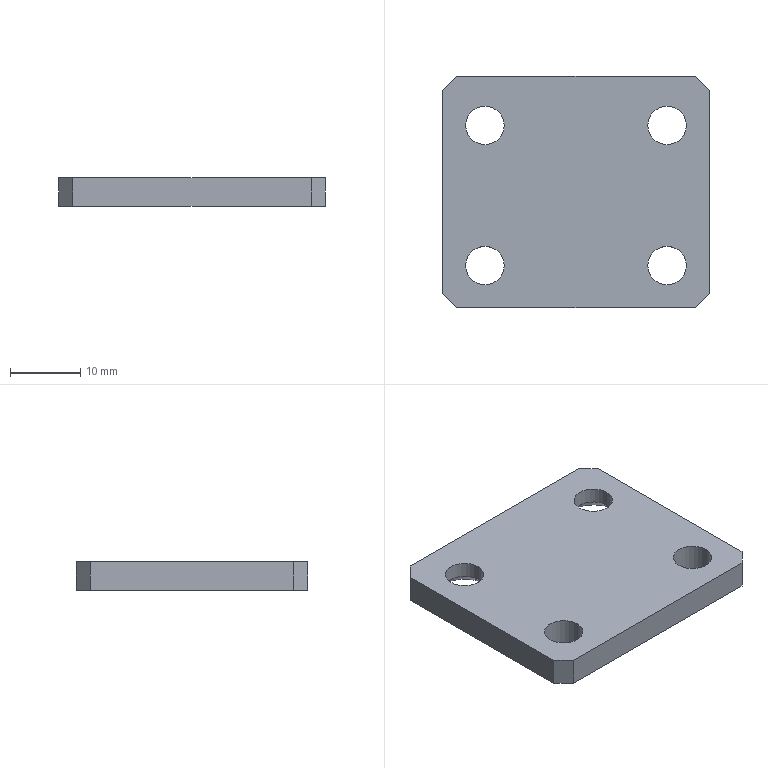Component | SolidWorks | DZ.KX.203-TC1505-30-09-01-05-20-1 | 1 solid | 22 faces | box 38 x 33 x 4 mm | volume 4540 mm3 | plane 10 | cylinder 8 | cone 4 | commonest cylinder face diameters 5.5 x8
build123d program:
from build123d import *

# Parameters (mm, degrees)
SKETCH1_W                                    = 38
SKETCH1_H                                    = 33
BOSS_EXTRUDE1_DEPTH                          = 4
HOLE_SIZE_SLOTTED_RAISED_COUNTERSUNK_2_COUNT = 2
HOLE_SIZE_SLOTTED_RAISED_COUNTERSUNK_2_PITCH = 26
F_5_5_5_5_DIAMETER_HOLE1_D                   = 5.5
CHAMFER1_SIZE                                = 2


with BuildPart() as part:
    # Sketch1 → Boss-Extrude1 (new body)
    with BuildSketch(Plane.XY):
        Rectangle(SKETCH1_W, SKETCH1_H)
    extrude(amount=BOSS_EXTRUDE1_DEPTH)

    # Sketch2 → Hole Size Slotted Raised Countersunk Scr (revolve, cut)
    with BuildSketch(Plane(origin=(13, 9.5, 0), x_dir=(0, 1, 0), z_dir=(1, 0, 0))):
        Polygon((0, 0), (0, 4), (2.75, 4), (2.75, 1.75), (4.5, 0), align=None)
    hole_size_slotted_raised_countersunk_scr = revolve(axis=Axis((13, 9.5, -6.35), (0, 0, 1)), mode=Mode.SUBTRACT)

    # Hole Size Slotted Raised Countersunk 2: Hole Size Slotted Raised Countersunk Scr ×2
    with Locations(*[(-i * HOLE_SIZE_SLOTTED_RAISED_COUNTERSUNK_2_PITCH, 0, 0) for i in range(1, HOLE_SIZE_SLOTTED_RAISED_COUNTERSUNK_2_COUNT)]):
        add(hole_size_slotted_raised_countersunk_scr, mode=Mode.SUBTRACT)

    # 5.5 _5.5_ Diameter Hole1 (through all)
    with Locations(Plane(origin=(0, 0, 0), x_dir=(-1, 0, 0), z_dir=(0, 0, -1))):
        with Locations((-13, -10.5), (13, -10.5)):
            Hole(F_5_5_5_5_DIAMETER_HOLE1_D / 2)

    # Chamfer1
    chamfer1_edges = [part.edges().sort_by_distance(p)[0] for p in [
        (-19, 16.5, 2),
        (19, 16.5, 2),
        (19, -16.5, 2),
        (-19, -16.5, 2),
    ]]
    chamfer(chamfer1_edges, length=CHAMFER1_SIZE)


solid = part.part

# Placed as in the assembly
solid = solid.moved(Location((294.5, -584.807, 13.06), (0, 0, 0)))
STEP:
#1=COLOUR_RGB('',0.7922,0.8196,0.9333);
#2=FILL_AREA_STYLE_COLOUR('',#1);
#3=FILL_AREA_STYLE('',(#2));
#4=SURFACE_STYLE_FILL_AREA(#3);
#5=SURFACE_SIDE_STYLE('',(#4));
#6=SURFACE_STYLE_USAGE(.BOTH.,#5);
#7=PRESENTATION_STYLE_ASSIGNMENT((#6));
#8=CARTESIAN_POINT('',(12.215,-23.437,0.6716));
#9=VERTEX_POINT('',#8);
#10=CARTESIAN_POINT('',(11.998,-23.437,0.6716));
#11=VERTEX_POINT('',#10);
#12=CARTESIAN_POINT('',(12.106,-23.437,0.6716));
#13=DIRECTION('',(0.,0.,-1.));
#14=DIRECTION('',(-1.,0.,0.));
#15=AXIS2_PLACEMENT_3D('',#12,#13,#14);
#16=CIRCLE('',#15,0.1083);
#17=EDGE_CURVE('',#9,#11,#16,.T.);
#18=ORIENTED_EDGE('',*,*,#17,.F.);
#19=CARTESIAN_POINT('',(12.215,-23.437,0.5142));
#20=VERTEX_POINT('',#19);
#21=CARTESIAN_POINT('',(12.215,-23.437,0.5142));
#22=DIRECTION('',(0.,0.,-1.));
#23=VECTOR('',#22,39.37);
#24=LINE('',#21,#23);
#25=EDGE_CURVE('',#9,#20,#24,.T.);
#26=ORIENTED_EDGE('',*,*,#25,.T.);
#27=CARTESIAN_POINT('',(11.998,-23.437,0.5142));
#28=VERTEX_POINT('',#27);
#29=CARTESIAN_POINT('',(12.106,-23.437,0.5142));
#30=DIRECTION('',(0.,0.,-1.));
#31=DIRECTION('',(-1.,0.,0.));
#32=AXIS2_PLACEMENT_3D('',#29,#30,#31);
#33=CIRCLE('',#32,0.1083);
#34=EDGE_CURVE('',#20,#28,#33,.T.);
#35=ORIENTED_EDGE('',*,*,#34,.T.);
#36=CARTESIAN_POINT('',(11.998,-23.437,0.5142));
#37=DIRECTION('',(0.,0.,-1.));
#38=VECTOR('',#37,39.37);
#39=LINE('',#36,#38);
#40=EDGE_CURVE('',#11,#28,#39,.T.);
#41=ORIENTED_EDGE('',*,*,#40,.F.);
#42=EDGE_LOOP('',(#18,#26,#35,#41));
#43=FACE_OUTER_BOUND('',#42,.T.);
#44=CARTESIAN_POINT('',(12.106,-23.437,0.5142));
#45=DIRECTION('',(0.,0.,-1.));
#46=DIRECTION('',(-1.,0.,0.));
#47=AXIS2_PLACEMENT_3D('',#44,#45,#46);
#48=CYLINDRICAL_SURFACE('',#47,0.1083);
#49=ADVANCED_FACE('',(#43),#48,.F.);
#50=CARTESIAN_POINT('',(11.191,-23.437,0.6716));
#51=VERTEX_POINT('',#50);
#52=CARTESIAN_POINT('',(10.974,-23.437,0.6716));
#53=VERTEX_POINT('',#52);
#54=CARTESIAN_POINT('',(11.083,-23.437,0.6716));
#55=DIRECTION('',(0.,0.,-1.));
#56=DIRECTION('',(-1.,0.,0.));
#57=AXIS2_PLACEMENT_3D('',#54,#55,#56);
#58=CIRCLE('',#57,0.1083);
#59=EDGE_CURVE('',#51,#53,#58,.T.);
#60=ORIENTED_EDGE('',*,*,#59,.F.);
#61=CARTESIAN_POINT('',(11.191,-23.437,0.5142));
#62=VERTEX_POINT('',#61);
#63=CARTESIAN_POINT('',(11.191,-23.437,0.5142));
#64=DIRECTION('',(0.,0.,-1.));
#65=VECTOR('',#64,39.37);
#66=LINE('',#63,#65);
#67=EDGE_CURVE('',#51,#62,#66,.T.);
#68=ORIENTED_EDGE('',*,*,#67,.T.);
#69=CARTESIAN_POINT('',(10.974,-23.437,0.5142));
#70=VERTEX_POINT('',#69);
#71=CARTESIAN_POINT('',(11.083,-23.437,0.5142));
#72=DIRECTION('',(0.,0.,-1.));
#73=DIRECTION('',(-1.,0.,0.));
#74=AXIS2_PLACEMENT_3D('',#71,#72,#73);
#75=CIRCLE('',#74,0.1083);
#76=EDGE_CURVE('',#62,#70,#75,.T.);
#77=ORIENTED_EDGE('',*,*,#76,.T.);
#78=CARTESIAN_POINT('',(10.974,-23.437,0.5142));
#79=DIRECTION('',(0.,0.,-1.));
#80=VECTOR('',#79,39.37);
#81=LINE('',#78,#80);
#82=EDGE_CURVE('',#53,#70,#81,.T.);
#83=ORIENTED_EDGE('',*,*,#82,.F.);
#84=EDGE_LOOP('',(#60,#68,#77,#83));
#85=FACE_OUTER_BOUND('',#84,.T.);
#86=CARTESIAN_POINT('',(11.083,-23.437,0.5142));
#87=DIRECTION('',(0.,0.,-1.));
#88=DIRECTION('',(-1.,0.,0.));
#89=AXIS2_PLACEMENT_3D('',#86,#87,#88);
#90=CYLINDRICAL_SURFACE('',#89,0.1083);
#91=ADVANCED_FACE('',(#85),#90,.F.);
#92=CARTESIAN_POINT('',(12.215,-22.65,0.5831));
#93=VERTEX_POINT('',#92);
#94=CARTESIAN_POINT('',(11.998,-22.65,0.5831));
#95=VERTEX_POINT('',#94);
#96=CARTESIAN_POINT('',(12.106,-22.65,0.5831));
#97=DIRECTION('',(0.,0.,-1.));
#98=DIRECTION('',(-1.,0.,0.));
#99=AXIS2_PLACEMENT_3D('',#96,#97,#98);
#100=CIRCLE('',#99,0.1083);
#101=EDGE_CURVE('',#93,#95,#100,.T.);
#102=ORIENTED_EDGE('',*,*,#101,.F.);
#103=CARTESIAN_POINT('',(12.283,-22.65,0.5142));
#104=VERTEX_POINT('',#103);
#105=CARTESIAN_POINT('',(12.283,-22.65,0.5142));
#106=DIRECTION('',(0.7071,0.,-0.7071));
#107=VECTOR('',#106,39.37);
#108=LINE('',#105,#107);
#109=EDGE_CURVE('',#93,#104,#108,.T.);
#110=ORIENTED_EDGE('',*,*,#109,.T.);
#111=CARTESIAN_POINT('',(11.929,-22.65,0.5142));
#112=VERTEX_POINT('',#111);
#113=CARTESIAN_POINT('',(12.106,-22.65,0.5142));
#114=DIRECTION('',(0.,0.,-1.));
#115=DIRECTION('',(-1.,0.,0.));
#116=AXIS2_PLACEMENT_3D('',#113,#114,#115);
#117=CIRCLE('',#116,0.1772);
#118=EDGE_CURVE('',#104,#112,#117,.T.);
#119=ORIENTED_EDGE('',*,*,#118,.T.);
#120=CARTESIAN_POINT('',(11.929,-22.65,0.5142));
#121=DIRECTION('',(-0.7071,0.,-0.7071));
#122=VECTOR('',#121,39.37);
#123=LINE('',#120,#122);
#124=EDGE_CURVE('',#95,#112,#123,.T.);
#125=ORIENTED_EDGE('',*,*,#124,.F.);
#126=EDGE_LOOP('',(#102,#110,#119,#125));
#127=FACE_OUTER_BOUND('',#126,.T.);
#128=CARTESIAN_POINT('',(12.106,-22.65,0.5142));
#129=DIRECTION('',(0.,0.,-1.));
#130=DIRECTION('',(-1.,0.,0.));
#131=AXIS2_PLACEMENT_3D('',#128,#129,#130);
#132=CONICAL_SURFACE('',#131,0.1772,0.7854);
#133=ADVANCED_FACE('',(#127),#132,.F.);
#134=CARTESIAN_POINT('',(12.215,-22.65,0.6716));
#135=VERTEX_POINT('',#134);
#136=CARTESIAN_POINT('',(11.998,-22.65,0.6716));
#137=VERTEX_POINT('',#136);
#138=CARTESIAN_POINT('',(12.106,-22.65,0.6716));
#139=DIRECTION('',(0.,0.,-1.));
#140=DIRECTION('',(-1.,0.,0.));
#141=AXIS2_PLACEMENT_3D('',#138,#139,#140);
#142=CIRCLE('',#141,0.1083);
#143=EDGE_CURVE('',#135,#137,#142,.T.);
#144=ORIENTED_EDGE('',*,*,#143,.F.);
#145=CARTESIAN_POINT('',(12.215,-22.65,0.5142));
#146=DIRECTION('',(0.,0.,-1.));
#147=VECTOR('',#146,39.37);
#148=LINE('',#145,#147);
#149=EDGE_CURVE('',#135,#93,#148,.T.);
#150=ORIENTED_EDGE('',*,*,#149,.T.);
#151=ORIENTED_EDGE('',*,*,#101,.T.);
#152=CARTESIAN_POINT('',(11.998,-22.65,0.5142));
#153=DIRECTION('',(0.,0.,-1.));
#154=VECTOR('',#153,39.37);
#155=LINE('',#152,#154);
#156=EDGE_CURVE('',#137,#95,#155,.T.);
#157=ORIENTED_EDGE('',*,*,#156,.F.);
#158=EDGE_LOOP('',(#144,#150,#151,#157));
#159=FACE_OUTER_BOUND('',#158,.T.);
#160=CARTESIAN_POINT('',(12.106,-22.65,0.5142));
#161=DIRECTION('',(0.,0.,-1.));
#162=DIRECTION('',(-1.,0.,0.));
#163=AXIS2_PLACEMENT_3D('',#160,#161,#162);
#164=CYLINDRICAL_SURFACE('',#163,0.1083);
#165=ADVANCED_FACE('',(#159),#164,.F.);
#166=CARTESIAN_POINT('',(11.191,-22.65,0.5831));
#167=VERTEX_POINT('',#166);
#168=CARTESIAN_POINT('',(10.974,-22.65,0.5831));
#169=VERTEX_POINT('',#168);
#170=CARTESIAN_POINT('',(11.083,-22.65,0.5831));
#171=DIRECTION('',(0.,0.,-1.));
#172=DIRECTION('',(-1.,0.,0.));
#173=AXIS2_PLACEMENT_3D('',#170,#171,#172);
#174=CIRCLE('',#173,0.1083);
#175=EDGE_CURVE('',#167,#169,#174,.T.);
#176=ORIENTED_EDGE('',*,*,#175,.F.);
#177=CARTESIAN_POINT('',(11.26,-22.65,0.5142));
#178=VERTEX_POINT('',#177);
#179=CARTESIAN_POINT('',(11.26,-22.65,0.5142));
#180=DIRECTION('',(0.7071,0.,-0.7071));
#181=VECTOR('',#180,39.37);
#182=LINE('',#179,#181);
#183=EDGE_CURVE('',#167,#178,#182,.T.);
#184=ORIENTED_EDGE('',*,*,#183,.T.);
#185=CARTESIAN_POINT('',(10.906,-22.65,0.5142));
#186=VERTEX_POINT('',#185);
#187=CARTESIAN_POINT('',(11.083,-22.65,0.5142));
#188=DIRECTION('',(0.,0.,-1.));
#189=DIRECTION('',(-1.,0.,0.));
#190=AXIS2_PLACEMENT_3D('',#187,#188,#189);
#191=CIRCLE('',#190,0.1772);
#192=EDGE_CURVE('',#178,#186,#191,.T.);
#193=ORIENTED_EDGE('',*,*,#192,.T.);
#194=CARTESIAN_POINT('',(10.906,-22.65,0.5142));
#195=DIRECTION('',(-0.7071,0.,-0.7071));
#196=VECTOR('',#195,39.37);
#197=LINE('',#194,#196);
#198=EDGE_CURVE('',#169,#186,#197,.T.);
#199=ORIENTED_EDGE('',*,*,#198,.F.);
#200=EDGE_LOOP('',(#176,#184,#193,#199));
#201=FACE_OUTER_BOUND('',#200,.T.);
#202=CARTESIAN_POINT('',(11.083,-22.65,0.5142));
#203=DIRECTION('',(0.,0.,-1.));
#204=DIRECTION('',(-1.,0.,0.));
#205=AXIS2_PLACEMENT_3D('',#202,#203,#204);
#206=CONICAL_SURFACE('',#205,0.1772,0.7854);
#207=ADVANCED_FACE('',(#201),#206,.F.);
#208=CARTESIAN_POINT('',(11.191,-22.65,0.6716));
#209=VERTEX_POINT('',#208);
#210=CARTESIAN_POINT('',(10.974,-22.65,0.6716));
#211=VERTEX_POINT('',#210);
#212=CARTESIAN_POINT('',(11.083,-22.65,0.6716));
#213=DIRECTION('',(0.,0.,-1.));
#214=DIRECTION('',(-1.,0.,0.));
#215=AXIS2_PLACEMENT_3D('',#212,#213,#214);
#216=CIRCLE('',#215,0.1083);
#217=EDGE_CURVE('',#209,#211,#216,.T.);
#218=ORIENTED_EDGE('',*,*,#217,.F.);
#219=CARTESIAN_POINT('',(11.191,-22.65,0.5142));
#220=DIRECTION('',(0.,0.,-1.));
#221=VECTOR('',#220,39.37);
#222=LINE('',#219,#221);
#223=EDGE_CURVE('',#209,#167,#222,.T.);
#224=ORIENTED_EDGE('',*,*,#223,.T.);
#225=ORIENTED_EDGE('',*,*,#175,.T.);
#226=CARTESIAN_POINT('',(10.974,-22.65,0.5142));
#227=DIRECTION('',(0.,0.,-1.));
#228=VECTOR('',#227,39.37);
#229=LINE('',#226,#228);
#230=EDGE_CURVE('',#211,#169,#229,.T.);
#231=ORIENTED_EDGE('',*,*,#230,.F.);
#232=EDGE_LOOP('',(#218,#224,#225,#231));
#233=FACE_OUTER_BOUND('',#232,.T.);
#234=CARTESIAN_POINT('',(11.083,-22.65,0.5142));
#235=DIRECTION('',(0.,0.,-1.));
#236=DIRECTION('',(-1.,0.,0.));
#237=AXIS2_PLACEMENT_3D('',#234,#235,#236);
#238=CYLINDRICAL_SURFACE('',#237,0.1083);
#239=ADVANCED_FACE('',(#233),#238,.F.);
#240=CARTESIAN_POINT('',(10.846,-22.453,0.5142));
#241=VERTEX_POINT('',#240);
#242=CARTESIAN_POINT('',(10.846,-23.595,0.5142));
#243=VERTEX_POINT('',#242);
#244=CARTESIAN_POINT('',(10.846,-23.674,0.5142));
#245=DIRECTION('',(0.,-1.,0.));
#246=VECTOR('',#245,39.37);
#247=LINE('',#244,#246);
#248=EDGE_CURVE('',#241,#243,#247,.T.);
#249=ORIENTED_EDGE('',*,*,#248,.T.);
#250=CARTESIAN_POINT('',(10.846,-23.595,0.6716));
#251=VERTEX_POINT('',#250);
#252=CARTESIAN_POINT('',(10.846,-23.595,0.6716));
#253=DIRECTION('',(0.,0.,1.));
#254=VECTOR('',#253,39.37);
#255=LINE('',#252,#254);
#256=EDGE_CURVE('',#243,#251,#255,.T.);
#257=ORIENTED_EDGE('',*,*,#256,.T.);
#258=CARTESIAN_POINT('',(10.846,-22.453,0.6716));
#259=VERTEX_POINT('',#258);
#260=CARTESIAN_POINT('',(10.846,-23.674,0.6716));
#261=DIRECTION('',(0.,-1.,0.));
#262=VECTOR('',#261,39.37);
#263=LINE('',#260,#262);
#264=EDGE_CURVE('',#259,#251,#263,.T.);
#265=ORIENTED_EDGE('',*,*,#264,.F.);
#266=CARTESIAN_POINT('',(10.846,-22.453,0.6716));
#267=DIRECTION('',(0.,0.,-1.));
#268=VECTOR('',#267,39.37);
#269=LINE('',#266,#268);
#270=EDGE_CURVE('',#259,#241,#269,.T.);
#271=ORIENTED_EDGE('',*,*,#270,.T.);
#272=EDGE_LOOP('',(#249,#257,#265,#271));
#273=FACE_OUTER_BOUND('',#272,.T.);
#274=CARTESIAN_POINT('',(10.846,-23.674,0.6716));
#275=DIRECTION('',(1.,0.,0.));
#276=DIRECTION('',(0.,0.,-1.));
#277=AXIS2_PLACEMENT_3D('',#274,#275,#276);
#278=PLANE('',#277);
#279=ADVANCED_FACE('',(#273),#278,.F.);
#280=CARTESIAN_POINT('',(10.925,-23.674,0.5142));
#281=VERTEX_POINT('',#280);
#282=CARTESIAN_POINT('',(12.264,-23.674,0.5142));
#283=VERTEX_POINT('',#282);
#284=CARTESIAN_POINT('',(12.343,-23.674,0.5142));
#285=DIRECTION('',(1.,0.,0.));
#286=VECTOR('',#285,39.37);
#287=LINE('',#284,#286);
#288=EDGE_CURVE('',#281,#283,#287,.T.);
#289=ORIENTED_EDGE('',*,*,#288,.T.);
#290=CARTESIAN_POINT('',(12.264,-23.674,0.6716));
#291=VERTEX_POINT('',#290);
#292=CARTESIAN_POINT('',(12.264,-23.674,0.6716));
#293=DIRECTION('',(0.,0.,1.));
#294=VECTOR('',#293,39.37);
#295=LINE('',#292,#294);
#296=EDGE_CURVE('',#283,#291,#295,.T.);
#297=ORIENTED_EDGE('',*,*,#296,.T.);
#298=CARTESIAN_POINT('',(10.925,-23.674,0.6716));
#299=VERTEX_POINT('',#298);
#300=CARTESIAN_POINT('',(12.343,-23.674,0.6716));
#301=DIRECTION('',(1.,0.,0.));
#302=VECTOR('',#301,39.37);
#303=LINE('',#300,#302);
#304=EDGE_CURVE('',#299,#291,#303,.T.);
#305=ORIENTED_EDGE('',*,*,#304,.F.);
#306=CARTESIAN_POINT('',(10.925,-23.674,0.6716));
#307=DIRECTION('',(0.,0.,-1.));
#308=VECTOR('',#307,39.37);
#309=LINE('',#306,#308);
#310=EDGE_CURVE('',#299,#281,#309,.T.);
#311=ORIENTED_EDGE('',*,*,#310,.T.);
#312=EDGE_LOOP('',(#289,#297,#305,#311));
#313=FACE_OUTER_BOUND('',#312,.T.);
#314=CARTESIAN_POINT('',(12.343,-23.674,0.6716));
#315=DIRECTION('',(-0.,1.,0.));
#316=DIRECTION('',(-1.,-0.,0.));
#317=AXIS2_PLACEMENT_3D('',#314,#315,#316);
#318=PLANE('',#317);
#319=ADVANCED_FACE('',(#313),#318,.F.);
#320=CARTESIAN_POINT('',(12.343,-23.595,0.5142));
#321=VERTEX_POINT('',#320);
#322=CARTESIAN_POINT('',(12.343,-22.453,0.5142));
#323=VERTEX_POINT('',#322);
#324=CARTESIAN_POINT('',(12.343,-23.674,0.5142));
#325=DIRECTION('',(0.,1.,0.));
#326=VECTOR('',#325,39.37);
#327=LINE('',#324,#326);
#328=EDGE_CURVE('',#321,#323,#327,.T.);
#329=ORIENTED_EDGE('',*,*,#328,.T.);
#330=CARTESIAN_POINT('',(12.343,-22.453,0.6716));
#331=VERTEX_POINT('',#330);
#332=CARTESIAN_POINT('',(12.343,-22.453,0.6716));
#333=DIRECTION('',(0.,0.,1.));
#334=VECTOR('',#333,39.37);
#335=LINE('',#332,#334);
#336=EDGE_CURVE('',#323,#331,#335,.T.);
#337=ORIENTED_EDGE('',*,*,#336,.T.);
#338=CARTESIAN_POINT('',(12.343,-23.595,0.6716));
#339=VERTEX_POINT('',#338);
#340=CARTESIAN_POINT('',(12.343,-23.674,0.6716));
#341=DIRECTION('',(0.,1.,0.));
#342=VECTOR('',#341,39.37);
#343=LINE('',#340,#342);
#344=EDGE_CURVE('',#339,#331,#343,.T.);
#345=ORIENTED_EDGE('',*,*,#344,.F.);
#346=CARTESIAN_POINT('',(12.343,-23.595,0.6716));
#347=DIRECTION('',(0.,0.,-1.));
#348=VECTOR('',#347,39.37);
#349=LINE('',#346,#348);
#350=EDGE_CURVE('',#339,#321,#349,.T.);
#351=ORIENTED_EDGE('',*,*,#350,.T.);
#352=EDGE_LOOP('',(#329,#337,#345,#351));
#353=FACE_OUTER_BOUND('',#352,.T.);
#354=CARTESIAN_POINT('',(12.343,-23.674,0.6716));
#355=DIRECTION('',(-1.,0.,0.));
#356=DIRECTION('',(0.,0.,1.));
#357=AXIS2_PLACEMENT_3D('',#354,#355,#356);
#358=PLANE('',#357);
#359=ADVANCED_FACE('',(#353),#358,.F.);
#360=CARTESIAN_POINT('',(12.264,-22.374,0.6716));
#361=VERTEX_POINT('',#360);
#362=CARTESIAN_POINT('',(10.925,-22.374,0.6716));
#363=VERTEX_POINT('',#362);
#364=CARTESIAN_POINT('',(12.343,-22.374,0.6716));
#365=DIRECTION('',(-1.,-0.,0.));
#366=VECTOR('',#365,39.37);
#367=LINE('',#364,#366);
#368=EDGE_CURVE('',#361,#363,#367,.T.);
#369=ORIENTED_EDGE('',*,*,#368,.F.);
#370=CARTESIAN_POINT('',(12.264,-22.374,0.5142));
#371=VERTEX_POINT('',#370);
#372=CARTESIAN_POINT('',(12.264,-22.374,0.6716));
#373=DIRECTION('',(0.,0.,-1.));
#374=VECTOR('',#373,39.37);
#375=LINE('',#372,#374);
#376=EDGE_CURVE('',#361,#371,#375,.T.);
#377=ORIENTED_EDGE('',*,*,#376,.T.);
#378=CARTESIAN_POINT('',(10.925,-22.374,0.5142));
#379=VERTEX_POINT('',#378);
#380=CARTESIAN_POINT('',(12.343,-22.374,0.5142));
#381=DIRECTION('',(-1.,-0.,0.));
#382=VECTOR('',#381,39.37);
#383=LINE('',#380,#382);
#384=EDGE_CURVE('',#371,#379,#383,.T.);
#385=ORIENTED_EDGE('',*,*,#384,.T.);
#386=CARTESIAN_POINT('',(10.925,-22.374,0.6716));
#387=DIRECTION('',(0.,0.,1.));
#388=VECTOR('',#387,39.37);
#389=LINE('',#386,#388);
#390=EDGE_CURVE('',#379,#363,#389,.T.);
#391=ORIENTED_EDGE('',*,*,#390,.T.);
#392=EDGE_LOOP('',(#369,#377,#385,#391));
#393=FACE_OUTER_BOUND('',#392,.T.);
#394=CARTESIAN_POINT('',(12.343,-22.374,0.6716));
#395=DIRECTION('',(0.,-1.,0.));
#396=DIRECTION('',(1.,0.,0.));
#397=AXIS2_PLACEMENT_3D('',#394,#395,#396);
#398=PLANE('',#397);
#399=ADVANCED_FACE('',(#393),#398,.F.);
#400=CARTESIAN_POINT('',(12.106,-23.437,0.6716));
#401=DIRECTION('',(0.,0.,-1.));
#402=DIRECTION('',(-1.,0.,0.));
#403=AXIS2_PLACEMENT_3D('',#400,#401,#402);
#404=CIRCLE('',#403,0.1083);
#405=EDGE_CURVE('',#11,#9,#404,.T.);
#406=ORIENTED_EDGE('',*,*,#405,.T.);
#407=ORIENTED_EDGE('',*,*,#17,.T.);
#408=EDGE_LOOP('',(#406,#407));
#409=FACE_BOUND('',#408,.T.);
#410=CARTESIAN_POINT('',(11.083,-23.437,0.6716));
#411=DIRECTION('',(0.,0.,-1.));
#412=DIRECTION('',(-1.,0.,0.));
#413=AXIS2_PLACEMENT_3D('',#410,#411,#412);
#414=CIRCLE('',#413,0.1083);
#415=EDGE_CURVE('',#53,#51,#414,.T.);
#416=ORIENTED_EDGE('',*,*,#415,.T.);
#417=ORIENTED_EDGE('',*,*,#59,.T.);
#418=EDGE_LOOP('',(#416,#417));
#419=FACE_BOUND('',#418,.T.);
#420=CARTESIAN_POINT('',(12.106,-22.65,0.6716));
#421=DIRECTION('',(0.,0.,-1.));
#422=DIRECTION('',(-1.,0.,0.));
#423=AXIS2_PLACEMENT_3D('',#420,#421,#422);
#424=CIRCLE('',#423,0.1083);
#425=EDGE_CURVE('',#137,#135,#424,.T.);
#426=ORIENTED_EDGE('',*,*,#425,.T.);
#427=ORIENTED_EDGE('',*,*,#143,.T.);
#428=EDGE_LOOP('',(#426,#427));
#429=FACE_BOUND('',#428,.T.);
#430=CARTESIAN_POINT('',(11.083,-22.65,0.6716));
#431=DIRECTION('',(0.,0.,-1.));
#432=DIRECTION('',(-1.,0.,0.));
#433=AXIS2_PLACEMENT_3D('',#430,#431,#432);
#434=CIRCLE('',#433,0.1083);
#435=EDGE_CURVE('',#211,#209,#434,.T.);
#436=ORIENTED_EDGE('',*,*,#435,.T.);
#437=ORIENTED_EDGE('',*,*,#217,.T.);
#438=EDGE_LOOP('',(#436,#437));
#439=FACE_BOUND('',#438,.T.);
#440=ORIENTED_EDGE('',*,*,#344,.T.);
#441=CARTESIAN_POINT('',(12.254,-22.364,0.6716));
#442=DIRECTION('',(-0.7071,0.7071,0.));
#443=VECTOR('',#442,39.37);
#444=LINE('',#441,#443);
#445=EDGE_CURVE('',#331,#361,#444,.T.);
#446=ORIENTED_EDGE('',*,*,#445,.T.);
#447=ORIENTED_EDGE('',*,*,#368,.T.);
#448=CARTESIAN_POINT('',(10.935,-22.364,0.6716));
#449=DIRECTION('',(-0.7071,-0.7071,0.));
#450=VECTOR('',#449,39.37);
#451=LINE('',#448,#450);
#452=EDGE_CURVE('',#363,#259,#451,.T.);
#453=ORIENTED_EDGE('',*,*,#452,.T.);
#454=ORIENTED_EDGE('',*,*,#264,.T.);
#455=CARTESIAN_POINT('',(10.935,-23.683,0.6716));
#456=DIRECTION('',(0.7071,-0.7071,0.));
#457=VECTOR('',#456,39.37);
#458=LINE('',#455,#457);
#459=EDGE_CURVE('',#251,#299,#458,.T.);
#460=ORIENTED_EDGE('',*,*,#459,.T.);
#461=ORIENTED_EDGE('',*,*,#304,.T.);
#462=CARTESIAN_POINT('',(12.254,-23.683,0.6716));
#463=DIRECTION('',(0.7071,0.7071,0.));
#464=VECTOR('',#463,39.37);
#465=LINE('',#462,#464);
#466=EDGE_CURVE('',#291,#339,#465,.T.);
#467=ORIENTED_EDGE('',*,*,#466,.T.);
#468=EDGE_LOOP('',(#440,#446,#447,#453,#454,#460,#461,#467));
#469=FACE_OUTER_BOUND('',#468,.T.);
#470=CARTESIAN_POINT('',(11.594,-23.024,0.6716));
#471=DIRECTION('',(0.,0.,1.));
#472=DIRECTION('',(1.,0.,0.));
#473=AXIS2_PLACEMENT_3D('',#470,#471,#472);
#474=PLANE('',#473);
#475=ADVANCED_FACE('',(#409,#419,#429,#439,#469),#474,.T.);
#476=CARTESIAN_POINT('',(12.106,-23.437,0.5142));
#477=DIRECTION('',(0.,0.,-1.));
#478=DIRECTION('',(-1.,0.,0.));
#479=AXIS2_PLACEMENT_3D('',#476,#477,#478);
#480=CIRCLE('',#479,0.1083);
#481=EDGE_CURVE('',#28,#20,#480,.T.);
#482=ORIENTED_EDGE('',*,*,#481,.F.);
#483=ORIENTED_EDGE('',*,*,#34,.F.);
#484=EDGE_LOOP('',(#482,#483));
#485=FACE_BOUND('',#484,.T.);
#486=CARTESIAN_POINT('',(11.083,-23.437,0.5142));
#487=DIRECTION('',(0.,0.,-1.));
#488=DIRECTION('',(-1.,0.,0.));
#489=AXIS2_PLACEMENT_3D('',#486,#487,#488);
#490=CIRCLE('',#489,0.1083);
#491=EDGE_CURVE('',#70,#62,#490,.T.);
#492=ORIENTED_EDGE('',*,*,#491,.F.);
#493=ORIENTED_EDGE('',*,*,#76,.F.);
#494=EDGE_LOOP('',(#492,#493));
#495=FACE_BOUND('',#494,.T.);
#496=CARTESIAN_POINT('',(12.106,-22.65,0.5142));
#497=DIRECTION('',(0.,0.,-1.));
#498=DIRECTION('',(-1.,0.,0.));
#499=AXIS2_PLACEMENT_3D('',#496,#497,#498);
#500=CIRCLE('',#499,0.1772);
#501=EDGE_CURVE('',#112,#104,#500,.T.);
#502=ORIENTED_EDGE('',*,*,#501,.F.);
#503=ORIENTED_EDGE('',*,*,#118,.F.);
#504=EDGE_LOOP('',(#502,#503));
#505=FACE_BOUND('',#504,.T.);
#506=CARTESIAN_POINT('',(11.083,-22.65,0.5142));
#507=DIRECTION('',(0.,0.,-1.));
#508=DIRECTION('',(-1.,0.,0.));
#509=AXIS2_PLACEMENT_3D('',#506,#507,#508);
#510=CIRCLE('',#509,0.1772);
#511=EDGE_CURVE('',#186,#178,#510,.T.);
#512=ORIENTED_EDGE('',*,*,#511,.F.);
#513=ORIENTED_EDGE('',*,*,#192,.F.);
#514=EDGE_LOOP('',(#512,#513));
#515=FACE_BOUND('',#514,.T.);
#516=ORIENTED_EDGE('',*,*,#384,.F.);
#517=CARTESIAN_POINT('',(12.264,-22.374,0.5142));
#518=DIRECTION('',(0.7071,-0.7071,0.));
#519=VECTOR('',#518,39.37);
#520=LINE('',#517,#519);
#521=EDGE_CURVE('',#371,#323,#520,.T.);
#522=ORIENTED_EDGE('',*,*,#521,.T.);
#523=ORIENTED_EDGE('',*,*,#328,.F.);
#524=CARTESIAN_POINT('',(12.343,-23.595,0.5142));
#525=DIRECTION('',(-0.7071,-0.7071,0.));
#526=VECTOR('',#525,39.37);
#527=LINE('',#524,#526);
#528=EDGE_CURVE('',#321,#283,#527,.T.);
#529=ORIENTED_EDGE('',*,*,#528,.T.);
#530=ORIENTED_EDGE('',*,*,#288,.F.);
#531=CARTESIAN_POINT('',(10.925,-23.674,0.5142));
#532=DIRECTION('',(-0.7071,0.7071,0.));
#533=VECTOR('',#532,39.37);
#534=LINE('',#531,#533);
#535=EDGE_CURVE('',#281,#243,#534,.T.);
#536=ORIENTED_EDGE('',*,*,#535,.T.);
#537=ORIENTED_EDGE('',*,*,#248,.F.);
#538=CARTESIAN_POINT('',(10.846,-22.453,0.5142));
#539=DIRECTION('',(0.7071,0.7071,0.));
#540=VECTOR('',#539,39.37);
#541=LINE('',#538,#540);
#542=EDGE_CURVE('',#241,#379,#541,.T.);
#543=ORIENTED_EDGE('',*,*,#542,.T.);
#544=EDGE_LOOP('',(#516,#522,#523,#529,#530,#536,#537,#543));
#545=FACE_OUTER_BOUND('',#544,.T.);
#546=CARTESIAN_POINT('',(11.594,-23.024,0.5142));
#547=DIRECTION('',(0.,0.,1.));
#548=DIRECTION('',(1.,0.,0.));
#549=AXIS2_PLACEMENT_3D('',#546,#547,#548);
#550=PLANE('',#549);
#551=ADVANCED_FACE('',(#485,#495,#505,#515,#545),#550,.F.);
#552=ORIENTED_EDGE('',*,*,#223,.F.);
#553=ORIENTED_EDGE('',*,*,#435,.F.);
#554=ORIENTED_EDGE('',*,*,#230,.T.);
#555=CARTESIAN_POINT('',(11.083,-22.65,0.5831));
#556=DIRECTION('',(0.,0.,-1.));
#557=DIRECTION('',(-1.,0.,0.));
#558=AXIS2_PLACEMENT_3D('',#555,#556,#557);
#559=CIRCLE('',#558,0.1083);
#560=EDGE_CURVE('',#169,#167,#559,.T.);
#561=ORIENTED_EDGE('',*,*,#560,.T.);
#562=EDGE_LOOP('',(#552,#553,#554,#561));
#563=FACE_OUTER_BOUND('',#562,.T.);
#564=CARTESIAN_POINT('',(11.083,-22.65,0.5142));
#565=DIRECTION('',(0.,0.,-1.));
#566=DIRECTION('',(-1.,0.,0.));
#567=AXIS2_PLACEMENT_3D('',#564,#565,#566);
#568=CYLINDRICAL_SURFACE('',#567,0.1083);
#569=ADVANCED_FACE('',(#563),#568,.F.);
#570=ORIENTED_EDGE('',*,*,#183,.F.);
#571=ORIENTED_EDGE('',*,*,#560,.F.);
#572=ORIENTED_EDGE('',*,*,#198,.T.);
#573=ORIENTED_EDGE('',*,*,#511,.T.);
#574=EDGE_LOOP('',(#570,#571,#572,#573));
#575=FACE_OUTER_BOUND('',#574,.T.);
#576=CARTESIAN_POINT('',(11.083,-22.65,0.5142));
#577=DIRECTION('',(0.,0.,-1.));
#578=DIRECTION('',(-1.,0.,0.));
#579=AXIS2_PLACEMENT_3D('',#576,#577,#578);
#580=CONICAL_SURFACE('',#579,0.1772,0.7854);
#581=ADVANCED_FACE('',(#575),#580,.F.);
#582=ORIENTED_EDGE('',*,*,#149,.F.);
#583=ORIENTED_EDGE('',*,*,#425,.F.);
#584=ORIENTED_EDGE('',*,*,#156,.T.);
#585=CARTESIAN_POINT('',(12.106,-22.65,0.5831));
#586=DIRECTION('',(0.,0.,-1.));
#587=DIRECTION('',(-1.,0.,0.));
#588=AXIS2_PLACEMENT_3D('',#585,#586,#587);
#589=CIRCLE('',#588,0.1083);
#590=EDGE_CURVE('',#95,#93,#589,.T.);
#591=ORIENTED_EDGE('',*,*,#590,.T.);
#592=EDGE_LOOP('',(#582,#583,#584,#591));
#593=FACE_OUTER_BOUND('',#592,.T.);
#594=CARTESIAN_POINT('',(12.106,-22.65,0.5142));
#595=DIRECTION('',(0.,0.,-1.));
#596=DIRECTION('',(-1.,0.,0.));
#597=AXIS2_PLACEMENT_3D('',#594,#595,#596);
#598=CYLINDRICAL_SURFACE('',#597,0.1083);
#599=ADVANCED_FACE('',(#593),#598,.F.);
#600=ORIENTED_EDGE('',*,*,#109,.F.);
#601=ORIENTED_EDGE('',*,*,#590,.F.);
#602=ORIENTED_EDGE('',*,*,#124,.T.);
#603=ORIENTED_EDGE('',*,*,#501,.T.);
#604=EDGE_LOOP('',(#600,#601,#602,#603));
#605=FACE_OUTER_BOUND('',#604,.T.);
#606=CARTESIAN_POINT('',(12.106,-22.65,0.5142));
#607=DIRECTION('',(0.,0.,-1.));
#608=DIRECTION('',(-1.,0.,0.));
#609=AXIS2_PLACEMENT_3D('',#606,#607,#608);
#610=CONICAL_SURFACE('',#609,0.1772,0.7854);
#611=ADVANCED_FACE('',(#605),#610,.F.);
#612=ORIENTED_EDGE('',*,*,#67,.F.);
#613=ORIENTED_EDGE('',*,*,#415,.F.);
#614=ORIENTED_EDGE('',*,*,#82,.T.);
#615=ORIENTED_EDGE('',*,*,#491,.T.);
#616=EDGE_LOOP('',(#612,#613,#614,#615));
#617=FACE_OUTER_BOUND('',#616,.T.);
#618=CARTESIAN_POINT('',(11.083,-23.437,0.5142));
#619=DIRECTION('',(0.,0.,-1.));
#620=DIRECTION('',(-1.,0.,0.));
#621=AXIS2_PLACEMENT_3D('',#618,#619,#620);
#622=CYLINDRICAL_SURFACE('',#621,0.1083);
#623=ADVANCED_FACE('',(#617),#622,.F.);
#624=ORIENTED_EDGE('',*,*,#25,.F.);
#625=ORIENTED_EDGE('',*,*,#405,.F.);
#626=ORIENTED_EDGE('',*,*,#40,.T.);
#627=ORIENTED_EDGE('',*,*,#481,.T.);
#628=EDGE_LOOP('',(#624,#625,#626,#627));
#629=FACE_OUTER_BOUND('',#628,.T.);
#630=CARTESIAN_POINT('',(12.106,-23.437,0.5142));
#631=DIRECTION('',(0.,0.,-1.));
#632=DIRECTION('',(-1.,0.,0.));
#633=AXIS2_PLACEMENT_3D('',#630,#631,#632);
#634=CYLINDRICAL_SURFACE('',#633,0.1083);
#635=ADVANCED_FACE('',(#629),#634,.F.);
#636=ORIENTED_EDGE('',*,*,#445,.F.);
#637=ORIENTED_EDGE('',*,*,#336,.F.);
#638=ORIENTED_EDGE('',*,*,#521,.F.);
#639=ORIENTED_EDGE('',*,*,#376,.F.);
#640=EDGE_LOOP('',(#636,#637,#638,#639));
#641=FACE_OUTER_BOUND('',#640,.T.);
#642=CARTESIAN_POINT('',(12.264,-22.374,0.6716));
#643=DIRECTION('',(-0.7071,-0.7071,0.));
#644=DIRECTION('',(0.,0.,-1.));
#645=AXIS2_PLACEMENT_3D('',#642,#643,#644);
#646=PLANE('',#645);
#647=ADVANCED_FACE('',(#641),#646,.F.);
#648=ORIENTED_EDGE('',*,*,#466,.F.);
#649=ORIENTED_EDGE('',*,*,#296,.F.);
#650=ORIENTED_EDGE('',*,*,#528,.F.);
#651=ORIENTED_EDGE('',*,*,#350,.F.);
#652=EDGE_LOOP('',(#648,#649,#650,#651));
#653=FACE_OUTER_BOUND('',#652,.T.);
#654=CARTESIAN_POINT('',(12.343,-23.595,0.6716));
#655=DIRECTION('',(-0.7071,0.7071,0.));
#656=DIRECTION('',(0.,0.,-1.));
#657=AXIS2_PLACEMENT_3D('',#654,#655,#656);
#658=PLANE('',#657);
#659=ADVANCED_FACE('',(#653),#658,.F.);
#660=ORIENTED_EDGE('',*,*,#459,.F.);
#661=ORIENTED_EDGE('',*,*,#256,.F.);
#662=ORIENTED_EDGE('',*,*,#535,.F.);
#663=ORIENTED_EDGE('',*,*,#310,.F.);
#664=EDGE_LOOP('',(#660,#661,#662,#663));
#665=FACE_OUTER_BOUND('',#664,.T.);
#666=CARTESIAN_POINT('',(10.925,-23.674,0.6716));
#667=DIRECTION('',(0.7071,0.7071,0.));
#668=DIRECTION('',(0.,0.,-1.));
#669=AXIS2_PLACEMENT_3D('',#666,#667,#668);
#670=PLANE('',#669);
#671=ADVANCED_FACE('',(#665),#670,.F.);
#672=ORIENTED_EDGE('',*,*,#452,.F.);
#673=ORIENTED_EDGE('',*,*,#390,.F.);
#674=ORIENTED_EDGE('',*,*,#542,.F.);
#675=ORIENTED_EDGE('',*,*,#270,.F.);
#676=EDGE_LOOP('',(#672,#673,#674,#675));
#677=FACE_OUTER_BOUND('',#676,.T.);
#678=CARTESIAN_POINT('',(10.846,-22.453,0.6716));
#679=DIRECTION('',(0.7071,-0.7071,0.));
#680=DIRECTION('',(0.,0.,-1.));
#681=AXIS2_PLACEMENT_3D('',#678,#679,#680);
#682=PLANE('',#681);
#683=ADVANCED_FACE('',(#677),#682,.F.);
#684=CLOSED_SHELL('',(#49,#91,#133,#165,#207,#239,#279,#319,#359,#399,#475,#551,#569,#581,#599,#611,#623,#635,#647,#659,#671,#683));
#685=MANIFOLD_SOLID_BREP('',#684);
#686=STYLED_ITEM('',(#7),#685);
#687=(LENGTH_UNIT()NAMED_UNIT(*)SI_UNIT($,.METRE.));
#688=LENGTH_MEASURE_WITH_UNIT(LENGTH_MEASURE(0.0254),#687);
#689=DIMENSIONAL_EXPONENTS(1.,0.,0.,0.,0.,0.,0.);
#690=(CONVERSION_BASED_UNIT('',#688)LENGTH_UNIT()NAMED_UNIT(#689));
#691=UNCERTAINTY_MEASURE_WITH_UNIT(LENGTH_MEASURE(0.00001),#690,'','');
#692=(NAMED_UNIT(*)PLANE_ANGLE_UNIT()SI_UNIT($,.RADIAN.));
#693=(NAMED_UNIT(*)SI_UNIT($,.STERADIAN.)SOLID_ANGLE_UNIT());
#694=(GEOMETRIC_REPRESENTATION_CONTEXT(3)GLOBAL_UNCERTAINTY_ASSIGNED_CONTEXT((#691))GLOBAL_UNIT_ASSIGNED_CONTEXT((#690,#692,#693))REPRESENTATION_CONTEXT('',''));
#695=MECHANICAL_DESIGN_GEOMETRIC_PRESENTATION_REPRESENTATION('',(#686),#694);
#696=PRESENTATION_LAYER_ASSIGNMENT('','',(#686));
#697=CARTESIAN_POINT('',(0.,0.,0.));
#698=DIRECTION('',(0.,0.,1.));
#699=DIRECTION('',(1.,0.,0.));
#700=AXIS2_PLACEMENT_3D('',#697,#698,#699);
#701=(LENGTH_UNIT()NAMED_UNIT(*)SI_UNIT($,.METRE.));
#702=LENGTH_MEASURE_WITH_UNIT(LENGTH_MEASURE(0.0254),#701);
#703=DIMENSIONAL_EXPONENTS(1.,0.,0.,0.,0.,0.,0.);
#704=(CONVERSION_BASED_UNIT('',#702)LENGTH_UNIT()NAMED_UNIT(#703));
#705=UNCERTAINTY_MEASURE_WITH_UNIT(LENGTH_MEASURE(0.00001),#704,'','');
#706=(NAMED_UNIT(*)PLANE_ANGLE_UNIT()SI_UNIT($,.RADIAN.));
#707=(NAMED_UNIT(*)SI_UNIT($,.STERADIAN.)SOLID_ANGLE_UNIT());
#708=(GEOMETRIC_REPRESENTATION_CONTEXT(3)GLOBAL_UNCERTAINTY_ASSIGNED_CONTEXT((#705))GLOBAL_UNIT_ASSIGNED_CONTEXT((#704,#706,#707))REPRESENTATION_CONTEXT('',''));
#709=ADVANCED_BREP_SHAPE_REPRESENTATION('',(#685,#700),#708);